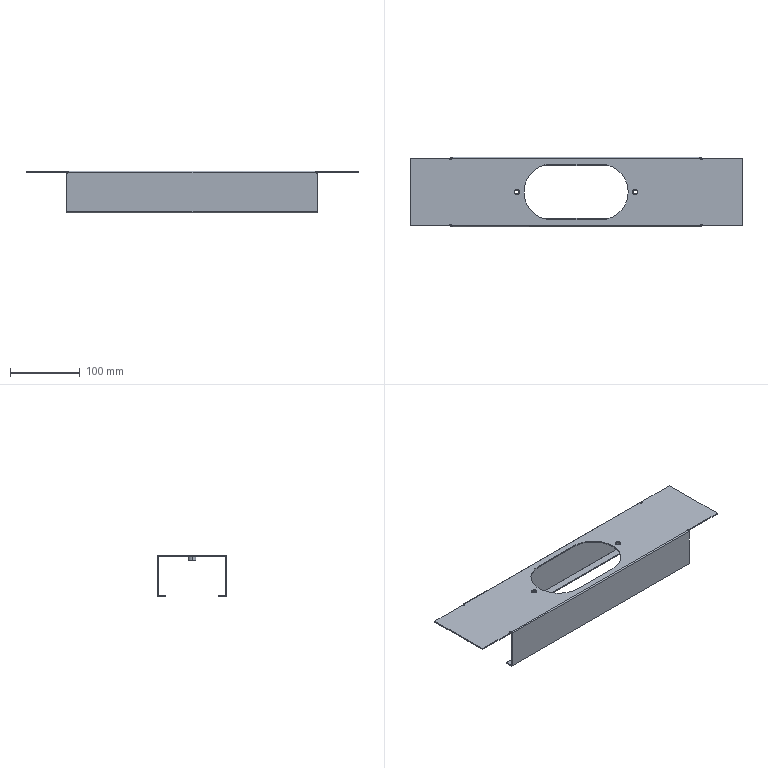Component | SolidWorks | BaseWeldment-1_BottomFrameLeftAndRight-1 | 1 solid | 79 faces | volume 129404 mm3 | plane 44 | cylinder 31 | spline 4 | commonest cylinder face diameters 4 x8 6 x4 11 x4 8 x4 0.2 x4 3.2 x4 80 x3